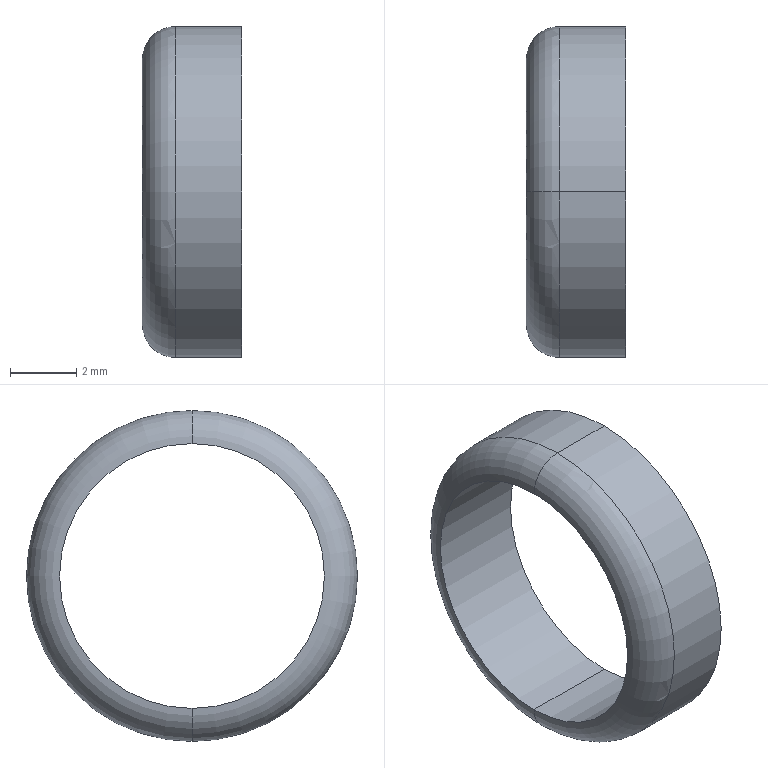Component | SolidWorks | PushRodFixingRing-1 | 1 solid | 7 faces | box 3 x 10 x 10 mm | volume 78 mm3 | cylinder 4 | torus 2 | plane 1 | commonest cylinder face diameters 8 x2 10 x2
STEP:
#1=COLOUR_RGB('',0.7922,0.8196,0.9333);
#2=FILL_AREA_STYLE_COLOUR('',#1);
#3=FILL_AREA_STYLE('',(#2));
#4=SURFACE_STYLE_FILL_AREA(#3);
#5=SURFACE_SIDE_STYLE('',(#4));
#6=SURFACE_STYLE_USAGE(.BOTH.,#5);
#7=PRESENTATION_STYLE_ASSIGNMENT((#6));
#8=CARTESIAN_POINT('',(1.207,8.661,-0.5906));
#9=VERTEX_POINT('',#8);
#10=CARTESIAN_POINT('',(1.207,8.661,-0.1969));
#11=VERTEX_POINT('',#10);
#12=CARTESIAN_POINT('',(1.207,8.661,-0.3937));
#13=DIRECTION('',(1.,0.,0.));
#14=DIRECTION('',(0.,0.,1.));
#15=AXIS2_PLACEMENT_3D('',#12,#13,#14);
#16=CIRCLE('',#15,0.1969);
#17=EDGE_CURVE('',#9,#11,#16,.T.);
#18=ORIENTED_EDGE('',*,*,#17,.F.);
#19=CARTESIAN_POINT('',(1.168,8.661,-0.5512));
#20=VERTEX_POINT('',#19);
#21=CARTESIAN_POINT('',(1.207,8.661,-0.5512));
#22=DIRECTION('',(-0.,1.,0.));
#23=DIRECTION('',(0.,0.,1.));
#24=AXIS2_PLACEMENT_3D('',#21,#22,#23);
#25=CIRCLE('',#24,0.03937);
#26=EDGE_CURVE('',#9,#20,#25,.T.);
#27=ORIENTED_EDGE('',*,*,#26,.T.);
#28=CARTESIAN_POINT('',(1.168,8.661,-0.2362));
#29=VERTEX_POINT('',#28);
#30=CARTESIAN_POINT('',(1.168,8.661,-0.3937));
#31=DIRECTION('',(-1.,-0.,-0.));
#32=DIRECTION('',(0.,0.,1.));
#33=AXIS2_PLACEMENT_3D('',#30,#31,#32);
#34=CIRCLE('',#33,0.1575);
#35=EDGE_CURVE('',#29,#20,#34,.T.);
#36=ORIENTED_EDGE('',*,*,#35,.F.);
#37=CARTESIAN_POINT('',(1.207,8.661,-0.2362));
#38=DIRECTION('',(0.,-1.,-0.));
#39=DIRECTION('',(0.,0.,-1.));
#40=AXIS2_PLACEMENT_3D('',#37,#38,#39);
#41=CIRCLE('',#40,0.03937);
#42=EDGE_CURVE('',#11,#29,#41,.T.);
#43=ORIENTED_EDGE('',*,*,#42,.F.);
#44=EDGE_LOOP('',(#18,#27,#36,#43));
#45=FACE_OUTER_BOUND('',#44,.T.);
#46=CARTESIAN_POINT('',(1.207,8.661,-0.3937));
#47=DIRECTION('',(-1.,-0.,-0.));
#48=DIRECTION('',(-0.,-0.,1.));
#49=AXIS2_PLACEMENT_3D('',#46,#47,#48);
#50=TOROIDAL_SURFACE('',#49,0.1575,0.03937);
#51=ADVANCED_FACE('',(#45),#50,.T.);
#52=CARTESIAN_POINT('',(1.168,8.661,-0.3937));
#53=DIRECTION('',(-1.,-0.,-0.));
#54=DIRECTION('',(0.,0.,1.));
#55=AXIS2_PLACEMENT_3D('',#52,#53,#54);
#56=CIRCLE('',#55,0.1575);
#57=EDGE_CURVE('',#20,#29,#56,.T.);
#58=ORIENTED_EDGE('',*,*,#57,.T.);
#59=CARTESIAN_POINT('',(1.286,8.661,-0.2362));
#60=VERTEX_POINT('',#59);
#61=CARTESIAN_POINT('',(1.168,8.661,-0.2362));
#62=DIRECTION('',(1.,0.,0.));
#63=VECTOR('',#62,39.37);
#64=LINE('',#61,#63);
#65=EDGE_CURVE('',#29,#60,#64,.T.);
#66=ORIENTED_EDGE('',*,*,#65,.T.);
#67=CARTESIAN_POINT('',(1.286,8.661,-0.5512));
#68=VERTEX_POINT('',#67);
#69=CARTESIAN_POINT('',(1.286,8.661,-0.3937));
#70=DIRECTION('',(-1.,-0.,-0.));
#71=DIRECTION('',(0.,0.,1.));
#72=AXIS2_PLACEMENT_3D('',#69,#70,#71);
#73=CIRCLE('',#72,0.1575);
#74=EDGE_CURVE('',#68,#60,#73,.T.);
#75=ORIENTED_EDGE('',*,*,#74,.F.);
#76=CARTESIAN_POINT('',(1.168,8.661,-0.5512));
#77=DIRECTION('',(1.,0.,0.));
#78=VECTOR('',#77,39.37);
#79=LINE('',#76,#78);
#80=EDGE_CURVE('',#20,#68,#79,.T.);
#81=ORIENTED_EDGE('',*,*,#80,.F.);
#82=EDGE_LOOP('',(#58,#66,#75,#81));
#83=FACE_OUTER_BOUND('',#82,.T.);
#84=CARTESIAN_POINT('',(1.168,8.661,-0.3937));
#85=DIRECTION('',(1.,0.,0.));
#86=DIRECTION('',(0.,0.,-1.));
#87=AXIS2_PLACEMENT_3D('',#84,#85,#86);
#88=CYLINDRICAL_SURFACE('',#87,0.1575);
#89=ADVANCED_FACE('',(#83),#88,.F.);
#90=ORIENTED_EDGE('',*,*,#17,.T.);
#91=CARTESIAN_POINT('',(1.286,8.661,-0.1969));
#92=VERTEX_POINT('',#91);
#93=CARTESIAN_POINT('',(1.168,8.661,-0.1969));
#94=DIRECTION('',(1.,0.,0.));
#95=VECTOR('',#94,39.37);
#96=LINE('',#93,#95);
#97=EDGE_CURVE('',#11,#92,#96,.T.);
#98=ORIENTED_EDGE('',*,*,#97,.T.);
#99=CARTESIAN_POINT('',(1.286,8.661,-0.5906));
#100=VERTEX_POINT('',#99);
#101=CARTESIAN_POINT('',(1.286,8.661,-0.3937));
#102=DIRECTION('',(-1.,-0.,-0.));
#103=DIRECTION('',(0.,0.,1.));
#104=AXIS2_PLACEMENT_3D('',#101,#102,#103);
#105=CIRCLE('',#104,0.1969);
#106=EDGE_CURVE('',#92,#100,#105,.T.);
#107=ORIENTED_EDGE('',*,*,#106,.T.);
#108=CARTESIAN_POINT('',(1.168,8.661,-0.5906));
#109=DIRECTION('',(1.,0.,0.));
#110=VECTOR('',#109,39.37);
#111=LINE('',#108,#110);
#112=EDGE_CURVE('',#9,#100,#111,.T.);
#113=ORIENTED_EDGE('',*,*,#112,.F.);
#114=EDGE_LOOP('',(#90,#98,#107,#113));
#115=FACE_OUTER_BOUND('',#114,.T.);
#116=CARTESIAN_POINT('',(1.168,8.661,-0.3937));
#117=DIRECTION('',(1.,0.,0.));
#118=DIRECTION('',(0.,0.,-1.));
#119=AXIS2_PLACEMENT_3D('',#116,#117,#118);
#120=CYLINDRICAL_SURFACE('',#119,0.1969);
#121=ADVANCED_FACE('',(#115),#120,.T.);
#122=CARTESIAN_POINT('',(1.286,8.661,-0.3937));
#123=DIRECTION('',(-1.,-0.,-0.));
#124=DIRECTION('',(0.,0.,1.));
#125=AXIS2_PLACEMENT_3D('',#122,#123,#124);
#126=CIRCLE('',#125,0.1969);
#127=EDGE_CURVE('',#100,#92,#126,.T.);
#128=ORIENTED_EDGE('',*,*,#127,.F.);
#129=ORIENTED_EDGE('',*,*,#106,.F.);
#130=EDGE_LOOP('',(#128,#129));
#131=FACE_OUTER_BOUND('',#130,.T.);
#132=ORIENTED_EDGE('',*,*,#74,.T.);
#133=CARTESIAN_POINT('',(1.286,8.661,-0.3937));
#134=DIRECTION('',(-1.,-0.,-0.));
#135=DIRECTION('',(0.,0.,1.));
#136=AXIS2_PLACEMENT_3D('',#133,#134,#135);
#137=CIRCLE('',#136,0.1575);
#138=EDGE_CURVE('',#60,#68,#137,.T.);
#139=ORIENTED_EDGE('',*,*,#138,.T.);
#140=EDGE_LOOP('',(#132,#139));
#141=FACE_BOUND('',#140,.T.);
#142=CARTESIAN_POINT('',(1.286,8.661,-0.3937));
#143=DIRECTION('',(-1.,-0.,-0.));
#144=DIRECTION('',(-0.,-0.,1.));
#145=AXIS2_PLACEMENT_3D('',#142,#143,#144);
#146=PLANE('',#145);
#147=ADVANCED_FACE('',(#131,#141),#146,.F.);
#148=ORIENTED_EDGE('',*,*,#97,.F.);
#149=CARTESIAN_POINT('',(1.207,8.661,-0.3937));
#150=DIRECTION('',(1.,0.,0.));
#151=DIRECTION('',(0.,0.,1.));
#152=AXIS2_PLACEMENT_3D('',#149,#150,#151);
#153=CIRCLE('',#152,0.1969);
#154=EDGE_CURVE('',#11,#9,#153,.T.);
#155=ORIENTED_EDGE('',*,*,#154,.T.);
#156=ORIENTED_EDGE('',*,*,#112,.T.);
#157=ORIENTED_EDGE('',*,*,#127,.T.);
#158=EDGE_LOOP('',(#148,#155,#156,#157));
#159=FACE_OUTER_BOUND('',#158,.T.);
#160=CARTESIAN_POINT('',(1.168,8.661,-0.3937));
#161=DIRECTION('',(1.,0.,0.));
#162=DIRECTION('',(0.,0.,-1.));
#163=AXIS2_PLACEMENT_3D('',#160,#161,#162);
#164=CYLINDRICAL_SURFACE('',#163,0.1969);
#165=ADVANCED_FACE('',(#159),#164,.T.);
#166=ORIENTED_EDGE('',*,*,#65,.F.);
#167=ORIENTED_EDGE('',*,*,#35,.T.);
#168=ORIENTED_EDGE('',*,*,#80,.T.);
#169=ORIENTED_EDGE('',*,*,#138,.F.);
#170=EDGE_LOOP('',(#166,#167,#168,#169));
#171=FACE_OUTER_BOUND('',#170,.T.);
#172=CARTESIAN_POINT('',(1.168,8.661,-0.3937));
#173=DIRECTION('',(1.,0.,0.));
#174=DIRECTION('',(0.,0.,-1.));
#175=AXIS2_PLACEMENT_3D('',#172,#173,#174);
#176=CYLINDRICAL_SURFACE('',#175,0.1575);
#177=ADVANCED_FACE('',(#171),#176,.F.);
#178=ORIENTED_EDGE('',*,*,#26,.F.);
#179=ORIENTED_EDGE('',*,*,#154,.F.);
#180=ORIENTED_EDGE('',*,*,#42,.T.);
#181=ORIENTED_EDGE('',*,*,#57,.F.);
#182=EDGE_LOOP('',(#178,#179,#180,#181));
#183=FACE_OUTER_BOUND('',#182,.T.);
#184=CARTESIAN_POINT('',(1.207,8.661,-0.3937));
#185=DIRECTION('',(-1.,-0.,-0.));
#186=DIRECTION('',(-0.,-0.,1.));
#187=AXIS2_PLACEMENT_3D('',#184,#185,#186);
#188=TOROIDAL_SURFACE('',#187,0.1575,0.03937);
#189=ADVANCED_FACE('',(#183),#188,.T.);
#190=CLOSED_SHELL('',(#51,#89,#121,#147,#165,#177,#189));
#191=MANIFOLD_SOLID_BREP('',#190);
#192=STYLED_ITEM('',(#7),#191);
#193=PRESENTATION_LAYER_ASSIGNMENT('','',(#192));
#194=(LENGTH_UNIT()NAMED_UNIT(*)SI_UNIT($,.METRE.));
#195=LENGTH_MEASURE_WITH_UNIT(LENGTH_MEASURE(0.0254),#194);
#196=DIMENSIONAL_EXPONENTS(1.,0.,0.,0.,0.,0.,0.);
#197=(CONVERSION_BASED_UNIT('',#195)LENGTH_UNIT()NAMED_UNIT(#196));
#198=UNCERTAINTY_MEASURE_WITH_UNIT(LENGTH_MEASURE(0.00001),#197,'','');
#199=(NAMED_UNIT(*)PLANE_ANGLE_UNIT()SI_UNIT($,.RADIAN.));
#200=(NAMED_UNIT(*)SI_UNIT($,.STERADIAN.)SOLID_ANGLE_UNIT());
#201=(GEOMETRIC_REPRESENTATION_CONTEXT(3)GLOBAL_UNCERTAINTY_ASSIGNED_CONTEXT((#198))GLOBAL_UNIT_ASSIGNED_CONTEXT((#197,#199,#200))REPRESENTATION_CONTEXT('',''));
#202=MECHANICAL_DESIGN_GEOMETRIC_PRESENTATION_REPRESENTATION('',(#192),#201);
#203=CARTESIAN_POINT('',(0.,0.,0.));
#204=DIRECTION('',(0.,0.,1.));
#205=DIRECTION('',(1.,0.,0.));
#206=AXIS2_PLACEMENT_3D('',#203,#204,#205);
#207=(LENGTH_UNIT()NAMED_UNIT(*)SI_UNIT($,.METRE.));
#208=LENGTH_MEASURE_WITH_UNIT(LENGTH_MEASURE(0.0254),#207);
#209=DIMENSIONAL_EXPONENTS(1.,0.,0.,0.,0.,0.,0.);
#210=(CONVERSION_BASED_UNIT('',#208)LENGTH_UNIT()NAMED_UNIT(#209));
#211=UNCERTAINTY_MEASURE_WITH_UNIT(LENGTH_MEASURE(0.00001),#210,'','');
#212=(NAMED_UNIT(*)PLANE_ANGLE_UNIT()SI_UNIT($,.RADIAN.));
#213=(NAMED_UNIT(*)SI_UNIT($,.STERADIAN.)SOLID_ANGLE_UNIT());
#214=(GEOMETRIC_REPRESENTATION_CONTEXT(3)GLOBAL_UNCERTAINTY_ASSIGNED_CONTEXT((#211))GLOBAL_UNIT_ASSIGNED_CONTEXT((#210,#212,#213))REPRESENTATION_CONTEXT('',''));
#215=ADVANCED_BREP_SHAPE_REPRESENTATION('',(#191,#206),#214);